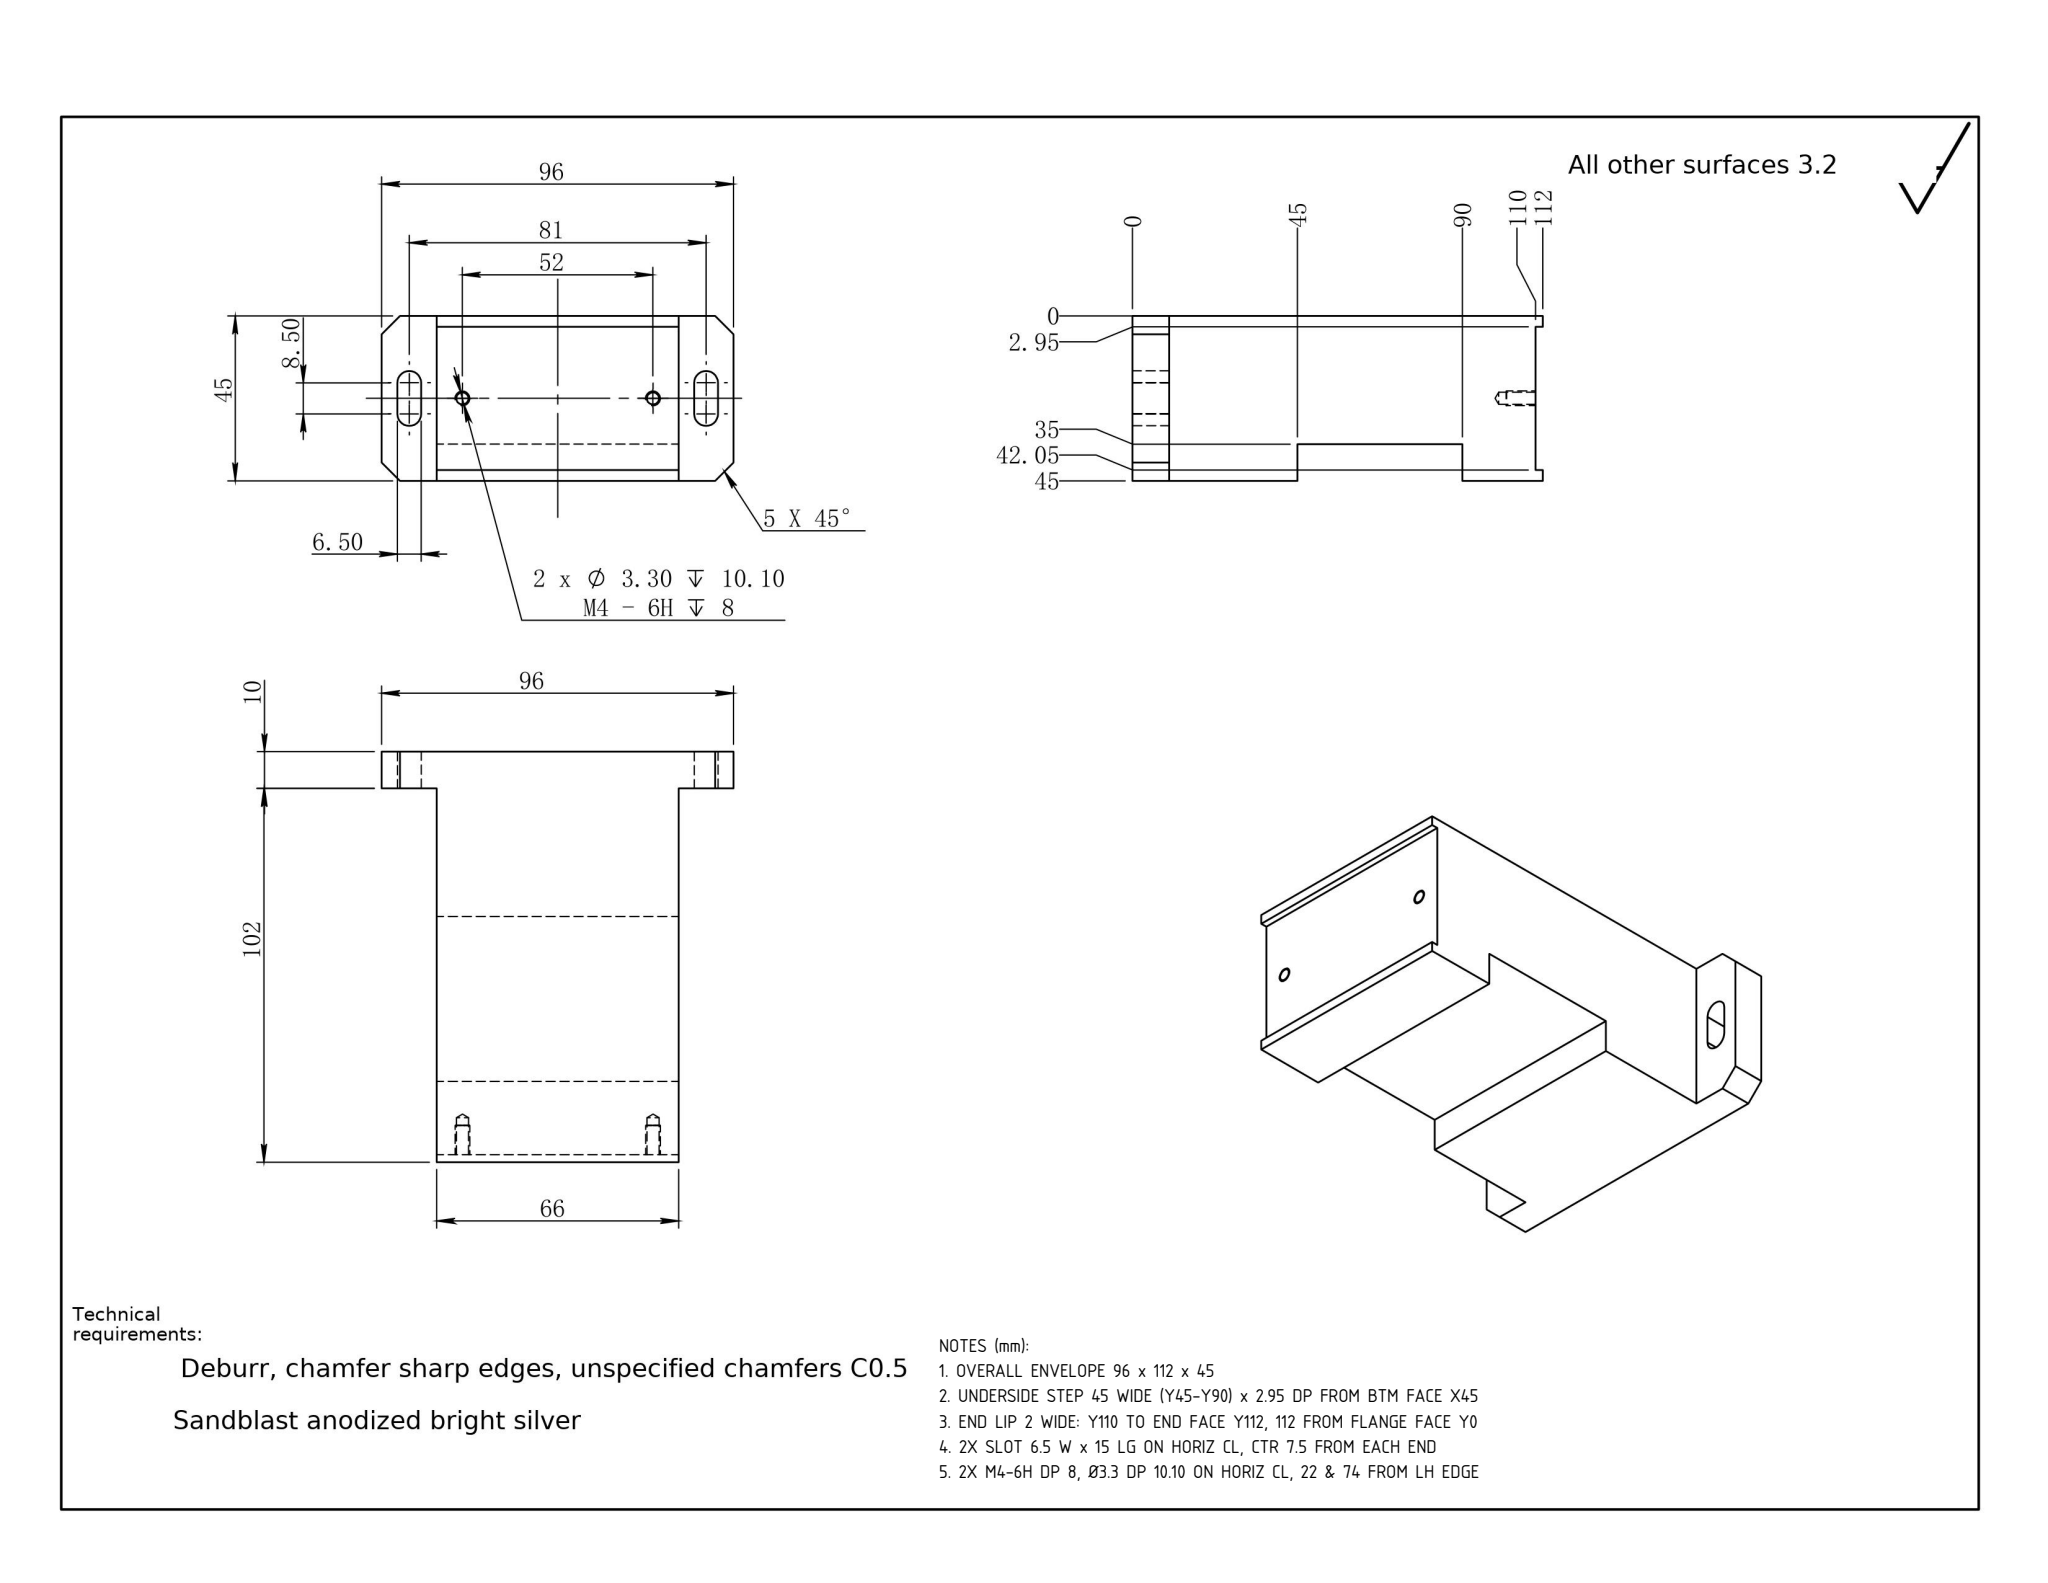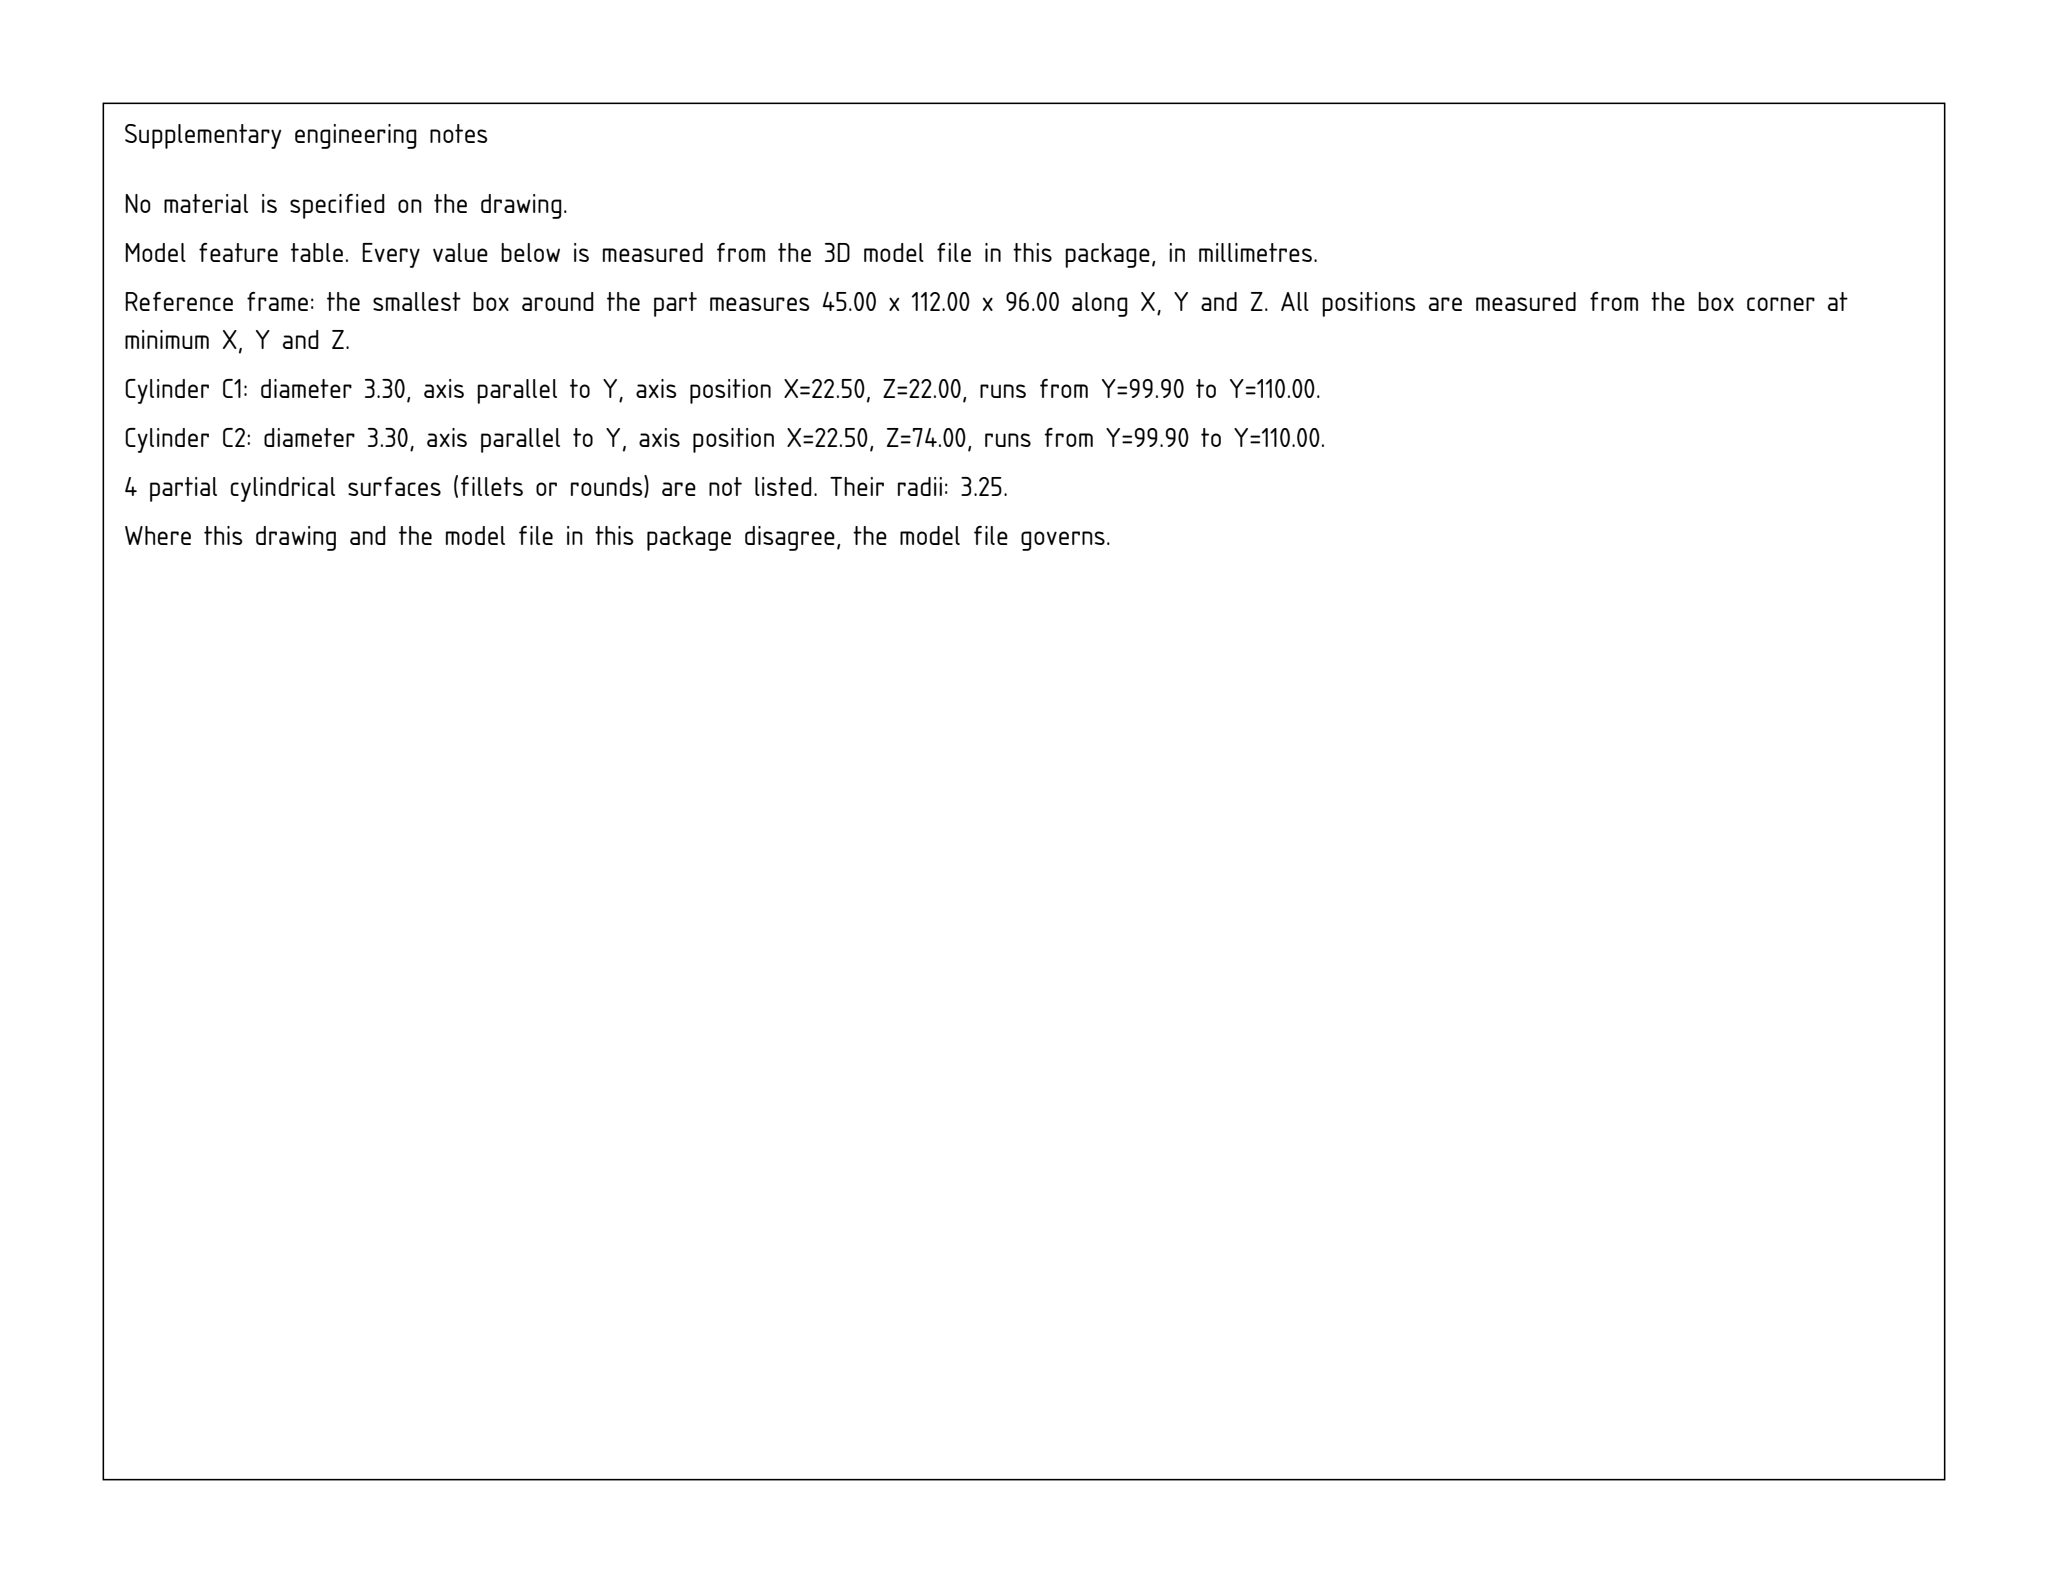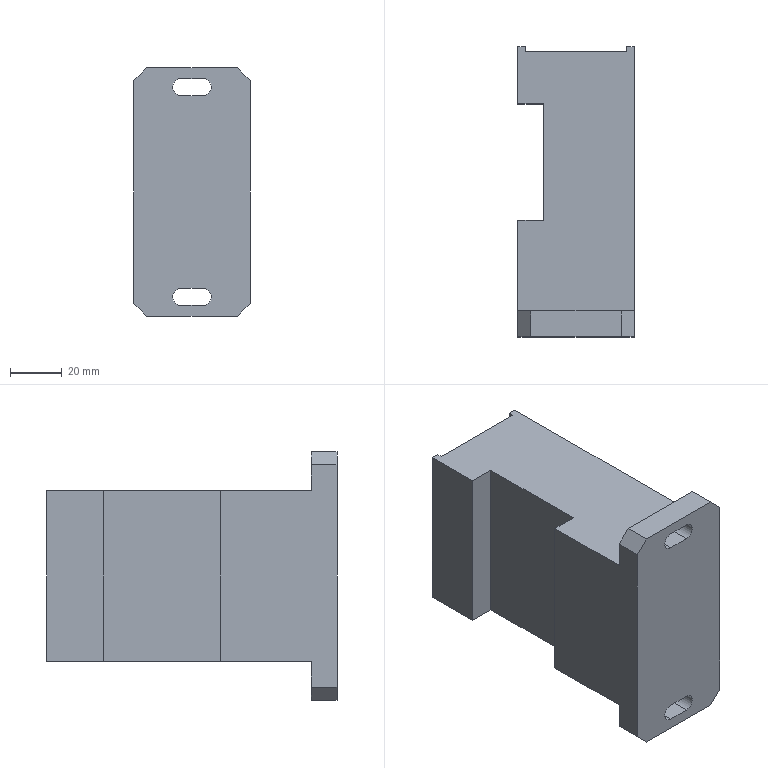Part | SolidWorks | mm | 1 solid | 38 faces | box 45 x 112 x 96 mm | volume 308832 mm3 | plane 26 | cylinder 8 | cone 4 | commonest cylinder face diameters 3.3 x4 6.5 x4
Drawing notes:
OVERALL ENVELOPE 96 x 112 x 45 | from the solid: bbox_xyz [45.0, 112.0, 96.0]
UNDERSIDE STEP 45 WIDE (Y45-Y90) x 2.95 DP FROM BTM FACE X45 | from the solid: y planes 45 and 90 (45 apart); x planes 42.05 and 45 -> 2.95 dp from bottom face x=45
END LIP 2 WIDE: Y110 TO END FACE Y112, 112 FROM FLANGE FACE Y0 | from the solid: y planes 110 and 112; bbox y = 112 from flange face y=0
2X SLOT 6.5 W x 15 LG ON HORIZ CL, CTR 7.5 FROM EACH END | from the solid: Ø6.5 y-cyls at z=7.5 and z=88.5 (96-88.5=7.5), x=18.25 & 26.75 -> 8.5 ctrs +6.5 = 15 lg; slot ctr x=22.5 = 45/2; z planes 4.25/10.75 and 85.25/91.75
2X M4-6H DP 8, Ø3.3 DP 10.10 ON HORIZ CL, 22 & 74 FROM LH EDGE | from the solid: Ø3.3 y-cyls at (x=22.5, z=22.0) and (x=22.5, z=74.0), L=10.1, 118° cone; x=22.5 = 45/2; 74-22=52